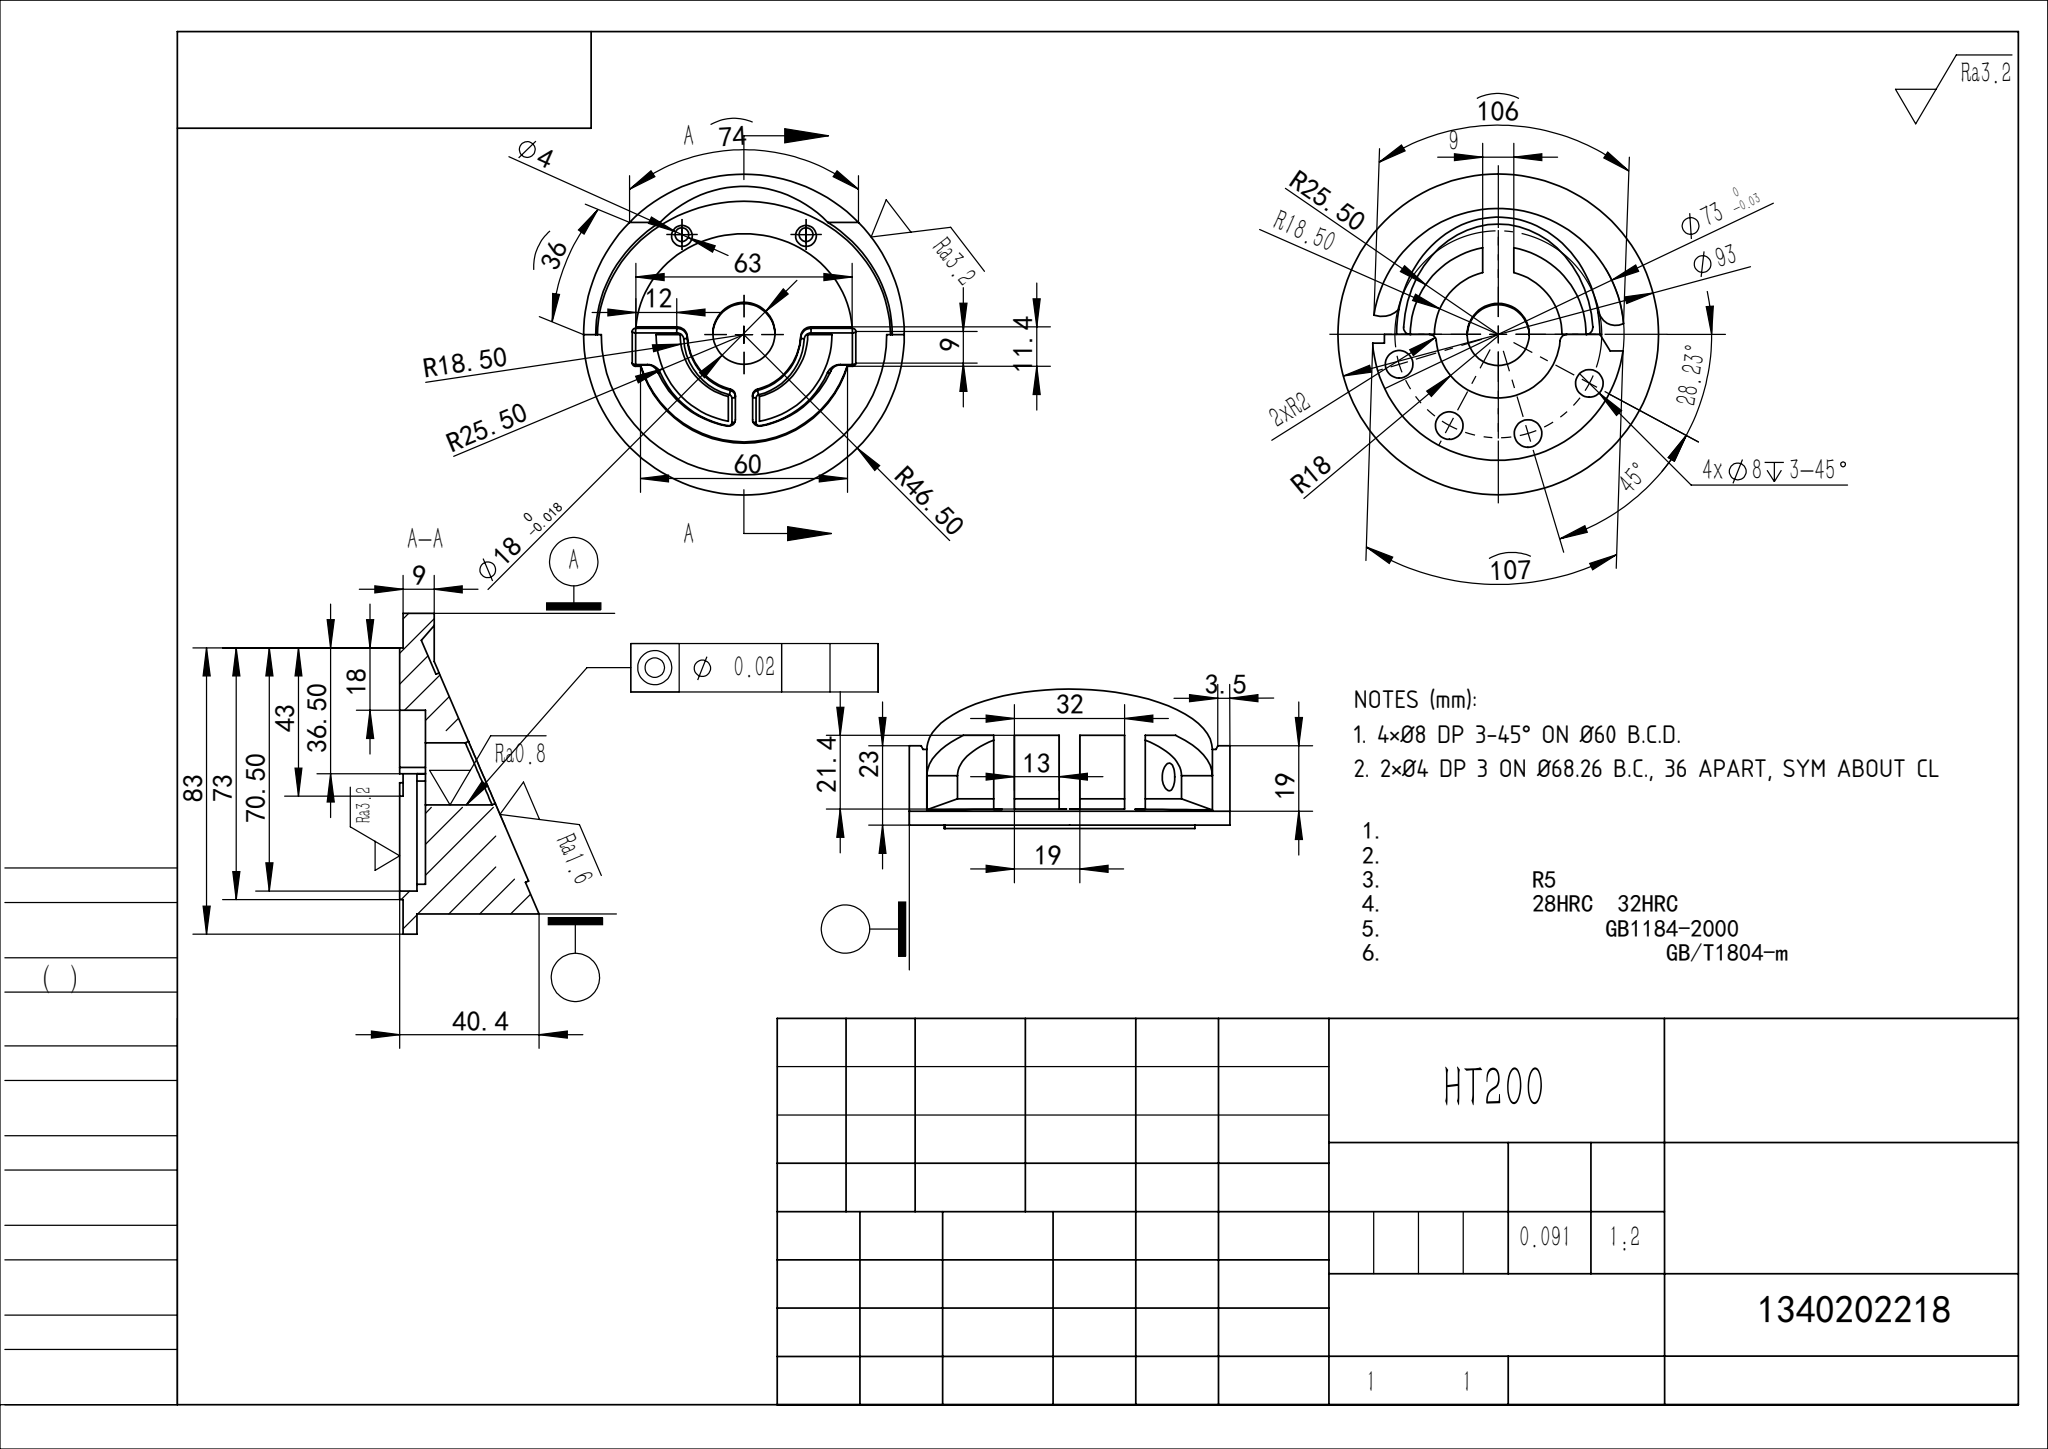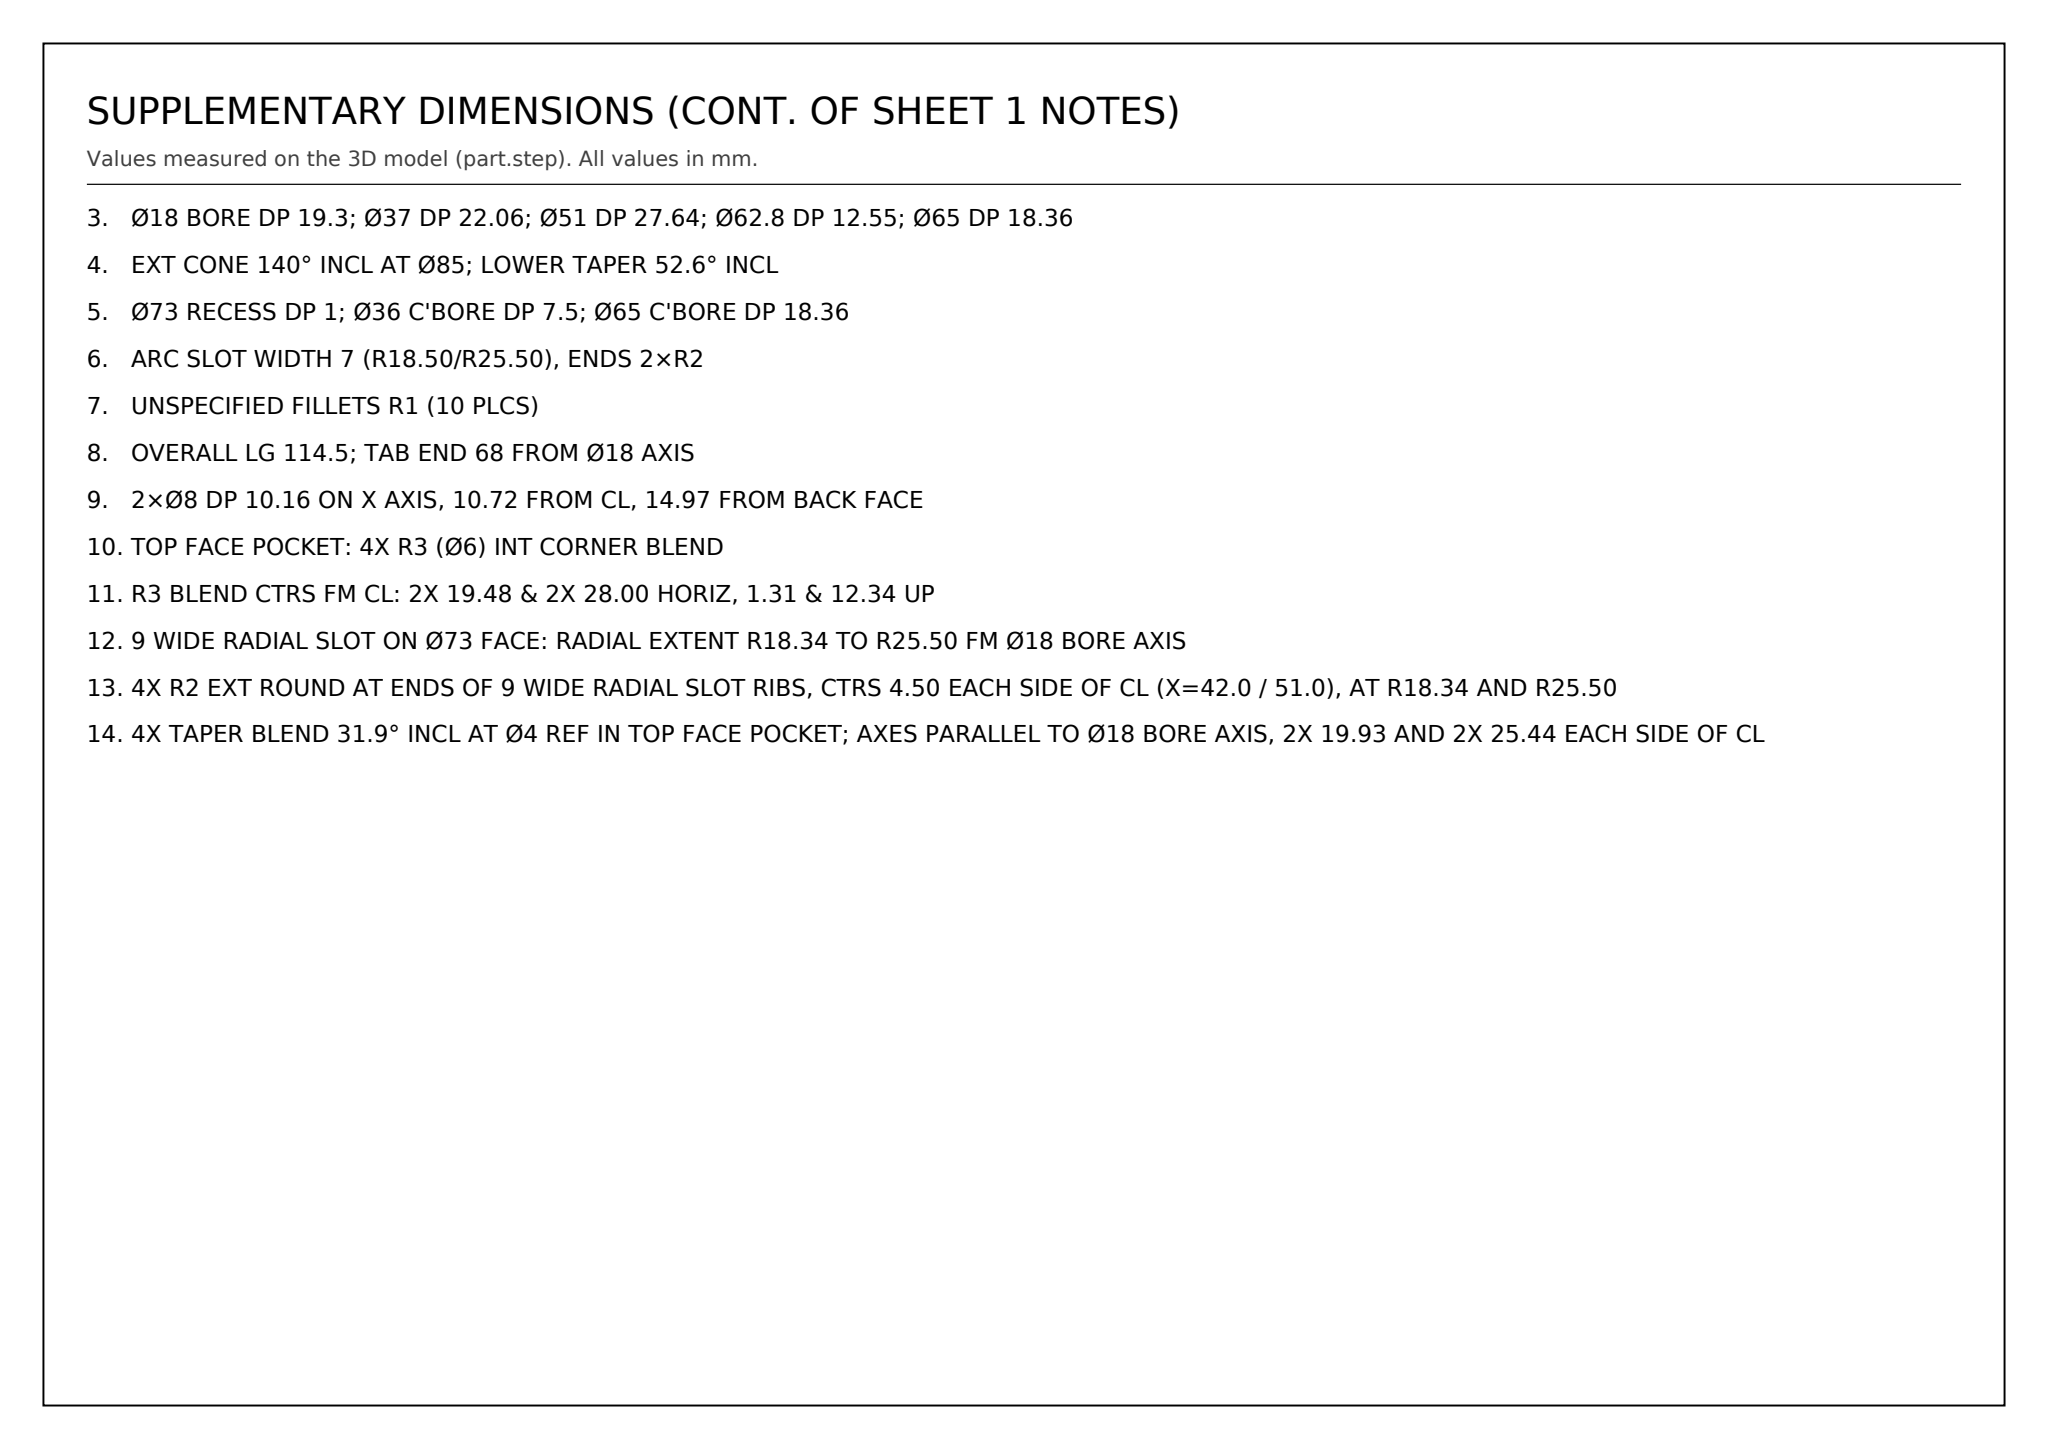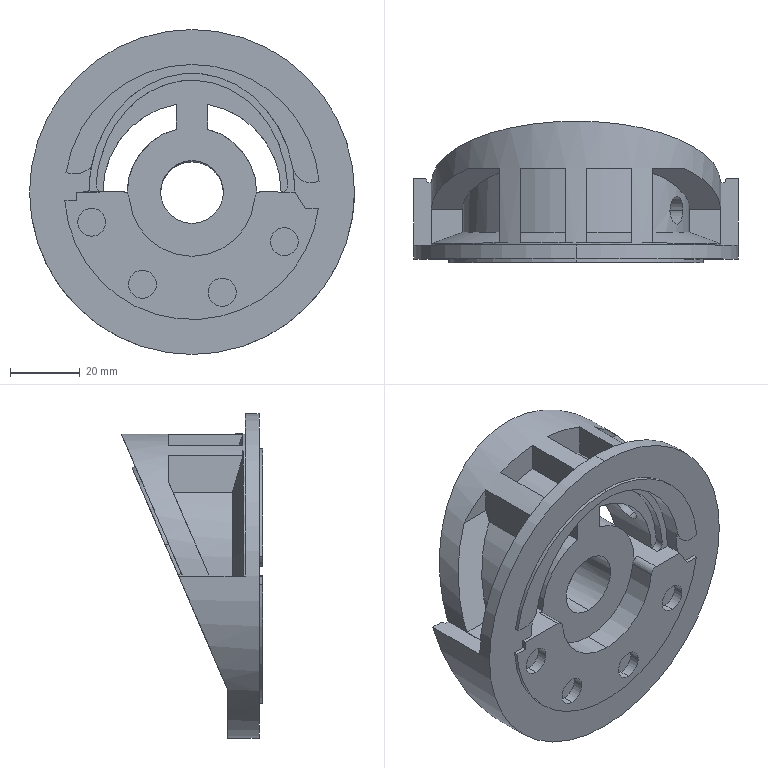Part | SolidWorks | mm | 1 solid | 150 faces | box 93 x 40.42 x 93 mm | volume 91354 mm3 | cylinder 57 | plane 53 | spline 16 | torus 10 | cone 9 | sphere 5 | commonest cylinder face diameters 4 x14 8 x10 2 x10 65 x4 6 x4 73 x3 36 x2 93 x2
Drawing notes:
4×Ø8 DP 3-45° ON Ø60 B.C.D. | from the solid: 4 Ø8 y-axis holes at (17.78,37.85),(32.31,20.07),(55.16,17.78),(72.93,32.31) = R30 from CL (46.5,46.5); depth 3.0
2×Ø4 DP 3 ON Ø68.26 B.C., 36 APART, SYM ABOUT CL | from the solid: Ø4 y-axis holes at x28.5 & x64.5, z17.5, len 3.0; ±18 from CL x46.5, 29 from CL z46.5 -> R34.13
Ø18 BORE DP 19.3; Ø37 DP 22.06; Ø51 DP 27.64; Ø62.8 DP 12.55; Ø65 DP 18.36 | from the solid: coaxial y cylinders at (46.5,46.5): Ø18 L19.3, Ø37 L22.06, Ø51 L27.64, Ø62.8 L12.55, Ø65 L18.36
EXT CONE 140° INCL AT Ø85; LOWER TAPER 52.6° INCL | from the solid: cones[included_angle,ref_dia]: [140.0,85.0] and [52.6,87.365]
Ø73 RECESS DP 1; Ø36 C'BORE DP 7.5; Ø65 C'BORE DP 18.36 | from the solid: Ø73 y cyl L1.0; Ø36 y cyl L7.5; Ø65 y cyl L18.36, all at (46.5,46.5)
ARC SLOT WIDTH 7 (R18.50/R25.50), ENDS 2×R2 | from the solid: R25.50-R18.50=7; 2×R2 slot-end radii per drawing, Ø4 end features at r20.03/r25.52
UNSPECIFIED FILLETS R1 (10 PLCS) | from the solid: fillet_radii: [[1.0,10]]
OVERALL LG 114.5; TAB END 68 FROM Ø18 AXIS | from the solid: bbox z=114.502; Ø18 axis at z46.5 -> 114.502-46.5=68.0
2×Ø8 DP 10.16 ON X AXIS, 10.72 FROM CL, 14.97 FROM BACK FACE | from the solid: cyl [8.0,'x',[null,14.97,57.22],10.16,2]; z57.22-46.5=10.72; y datum plane 0.0
TOP FACE POCKET: 4X R3 (Ø6) INT CORNER BLEND | from the solid: cylinders dia 6.0 axis y, 4 plcs: (18.5,58.84),(27.02,47.81),(65.98,47.81),(74.5,58.84)
R3 BLEND CTRS FM CL: 2X 19.48 & 2X 28.00 HORIZ, 1.31 & 12.34 UP | from the solid: part axis at x46.5,z46.5 (Ø93/Ø73 cyls); dx=±19.48,dz=+1.31 and dx=±28.00,dz=+12.34
9 WIDE RADIAL SLOT ON Ø73 FACE: RADIAL EXTENT R18.34 TO R25.50 FM Ø18 BORE AXIS | from the solid: Ø4 y-axis cylinders (R2 end rounds) at z=64.84 and z=72.00 vs bore axis at x=46.5, z=46.5 (18.0 dia y-axis cyl at [46.5,46.5])
4X R2 EXT ROUND AT ENDS OF 9 WIDE RADIAL SLOT RIBS, CTRS 4.50 EACH SIDE OF CL (X=42.0 / 51.0), AT R18.34 AND R25.50 | from the solid: cylinders [4.0,"y",[42.0,64.84]], [4.0,"y",[42.0,72.0]], [4.0,"y",[51.0,64.84]], [4.0,"y",[51.0,72.0]]
4X TAPER BLEND 31.9° INCL AT Ø4 REF IN TOP FACE POCKET; AXES PARALLEL TO Ø18 BORE AXIS, 2X 19.93 AND 2X 25.44 EACH SIDE OF CL | from the solid: cones [31.9, 4.0, 4]; Ø4 y-axis cylinders at x=26.57/66.44 (z=44.5) and x=21.06/71.94 (z=48.5), CL at x=46.5